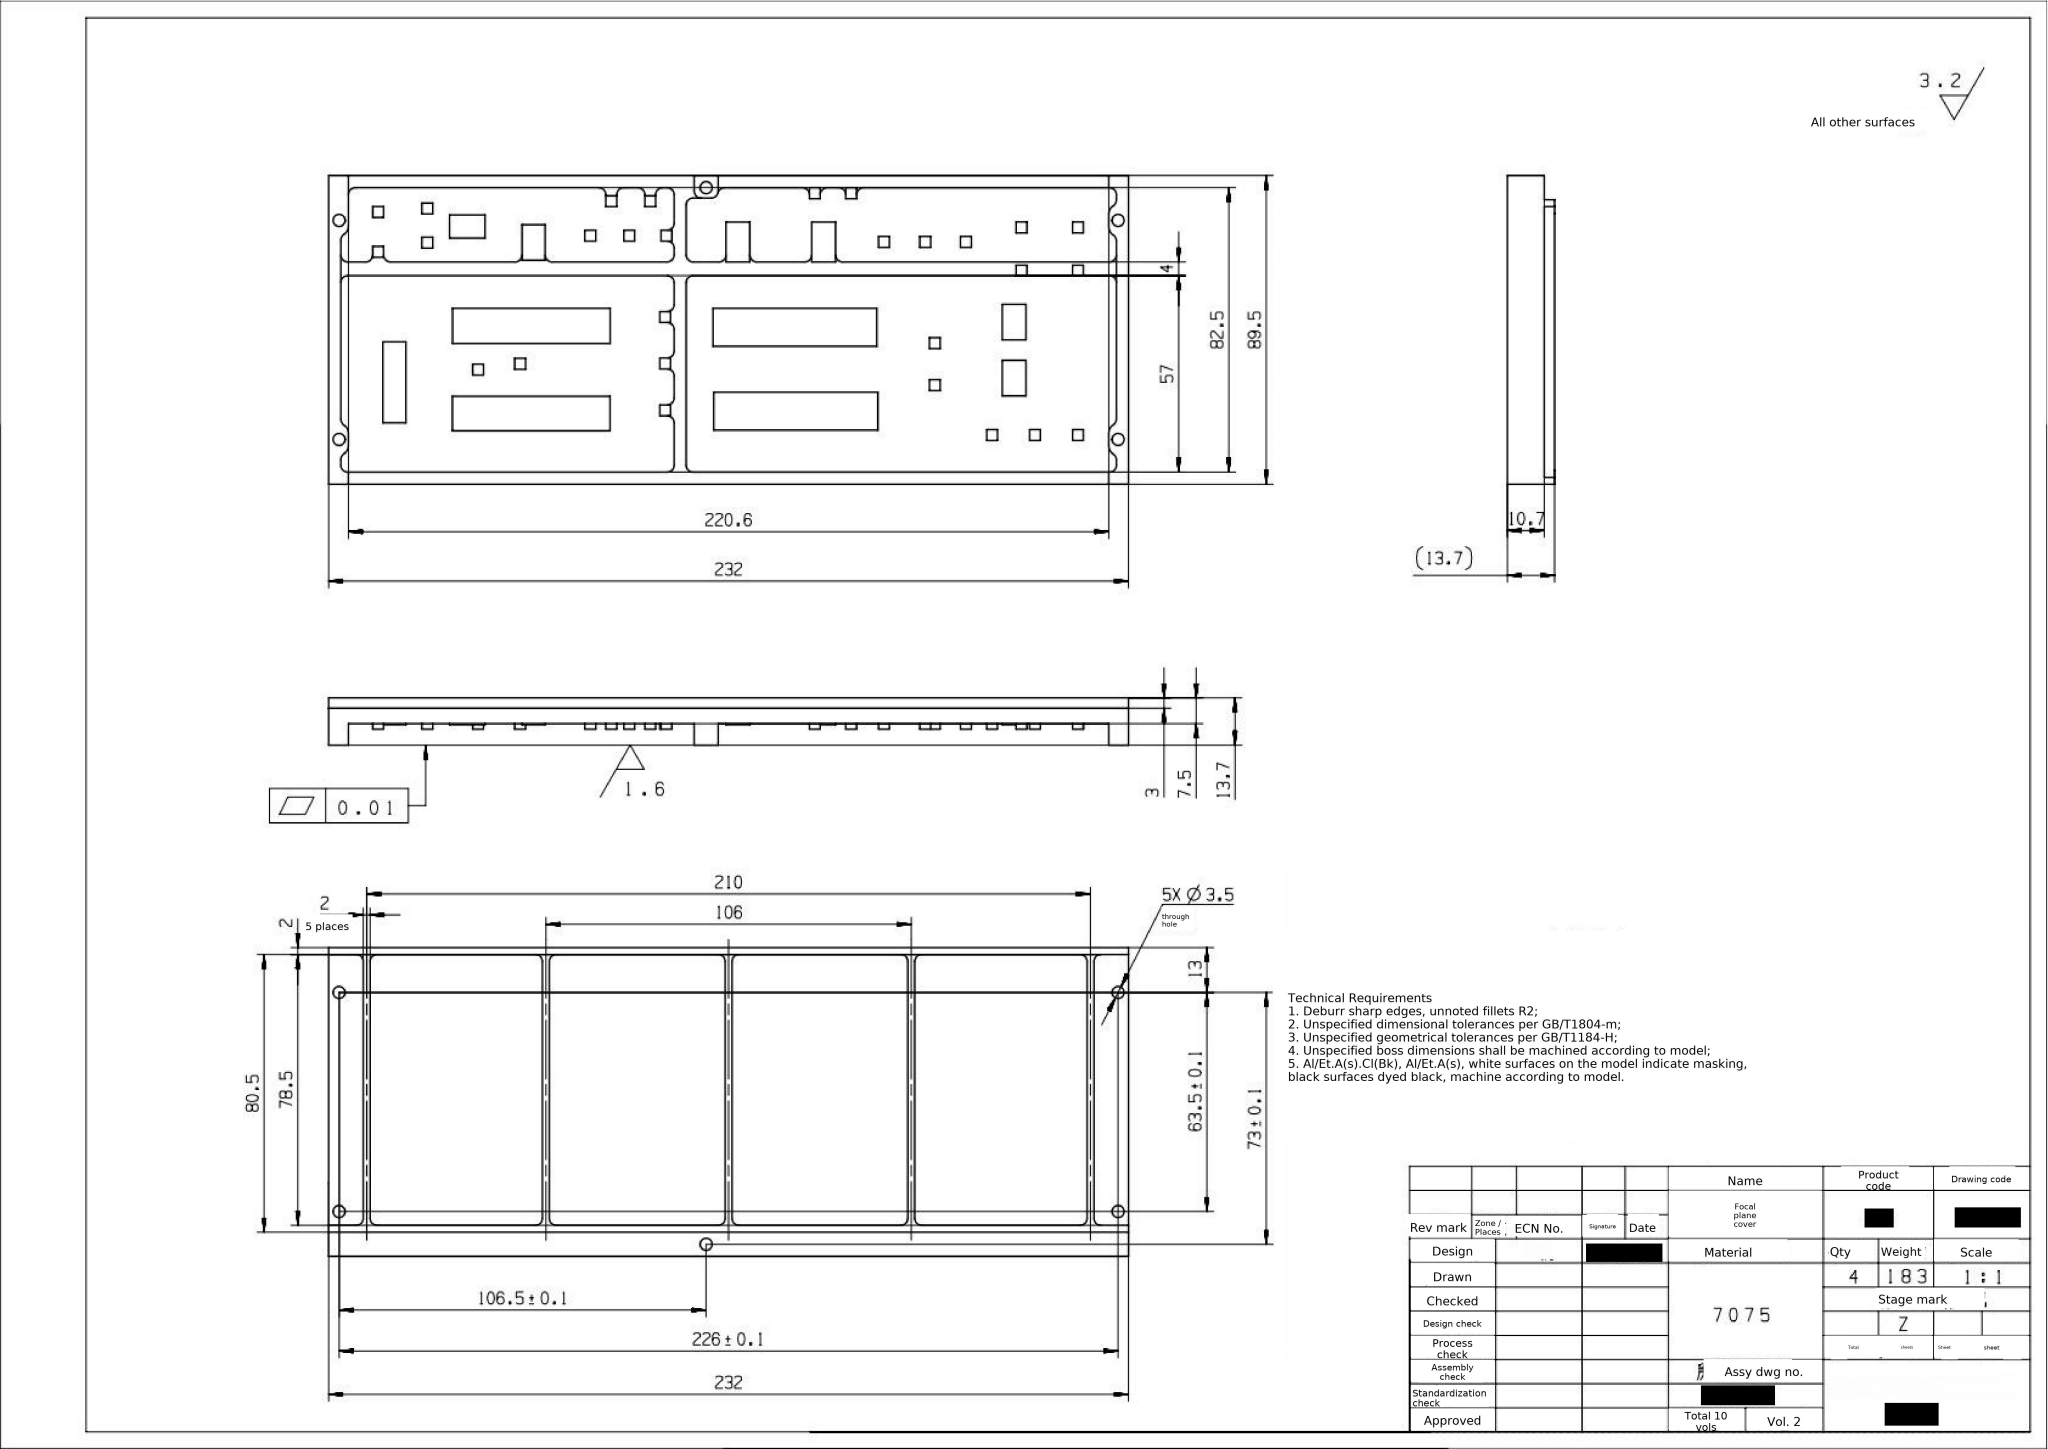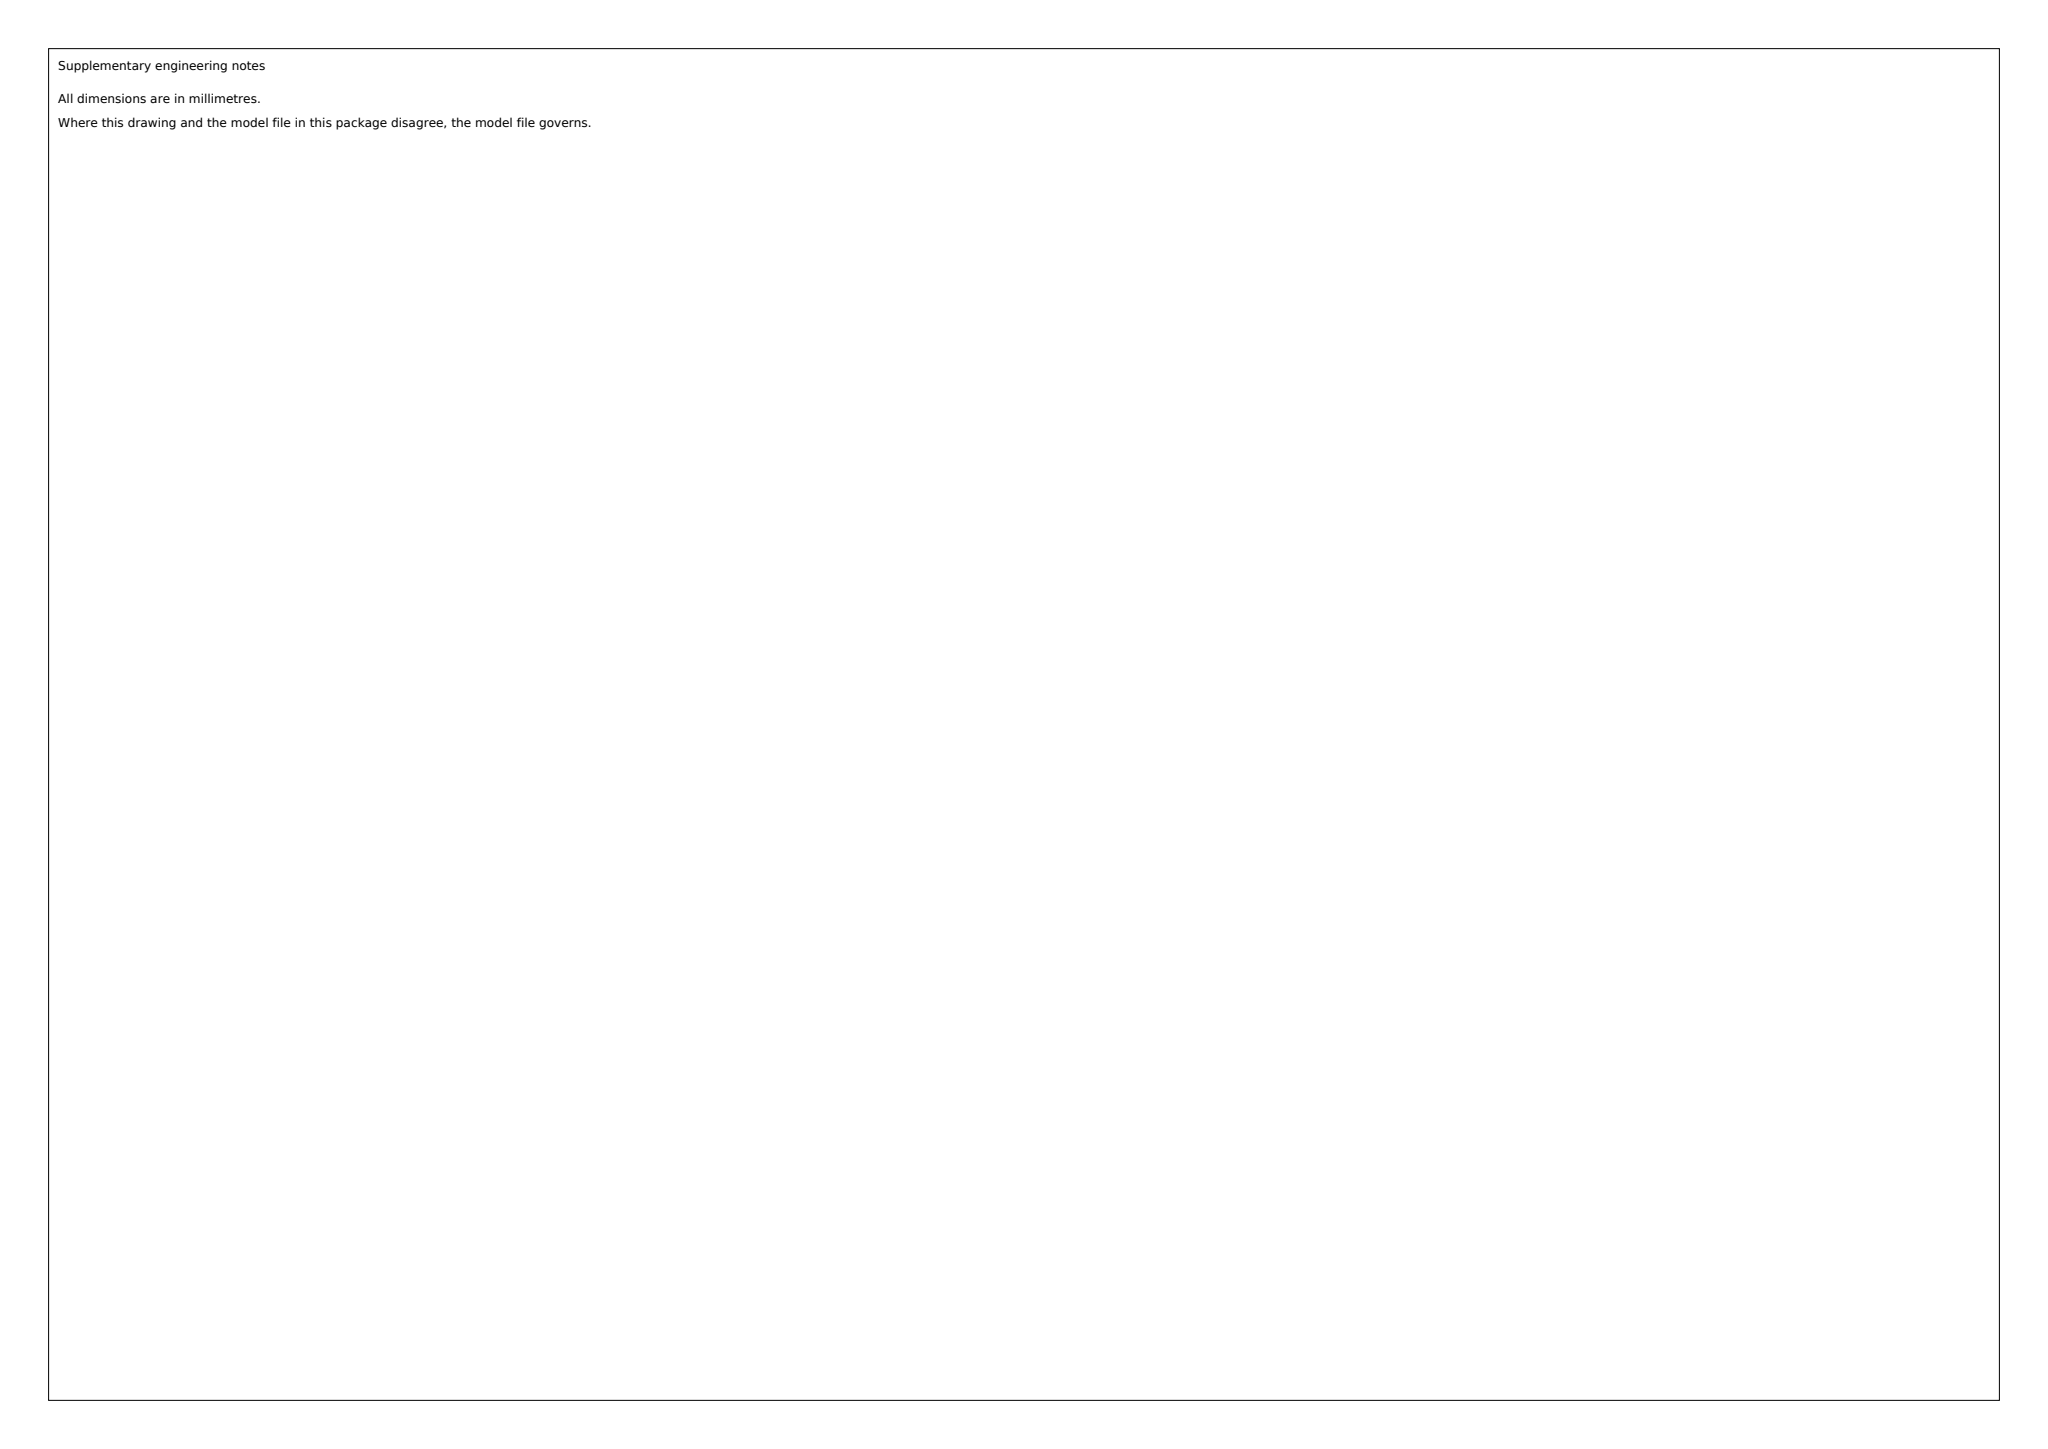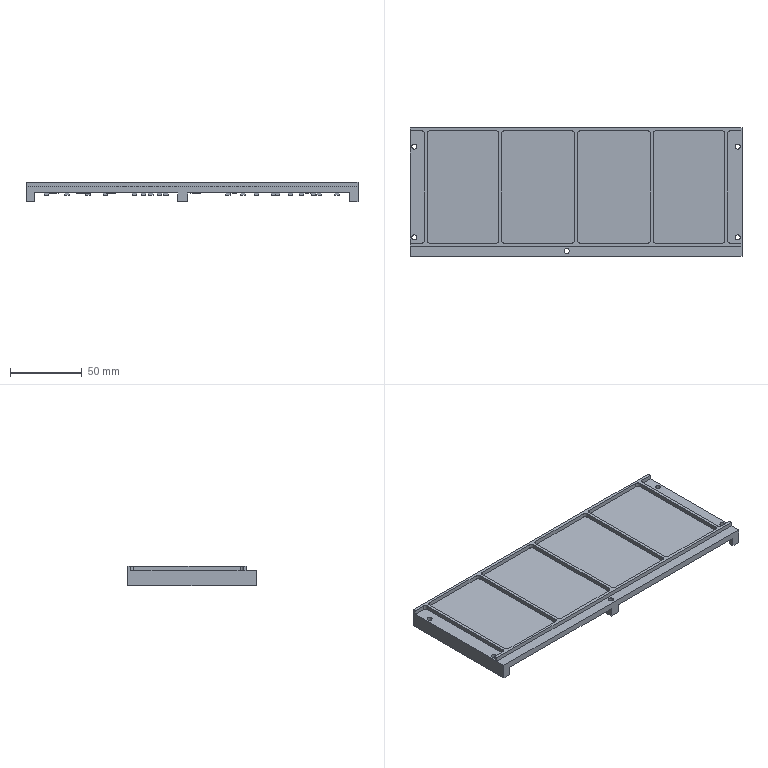Part | SolidWorks | mm | material 7075 | 1 solid | 364 faces | box 232 x 89.5 x 13.7 mm | volume 65870 mm3 | plane 277 | cylinder 87 | commonest cylinder face diameters 4 x70 3.5 x10 6 x7